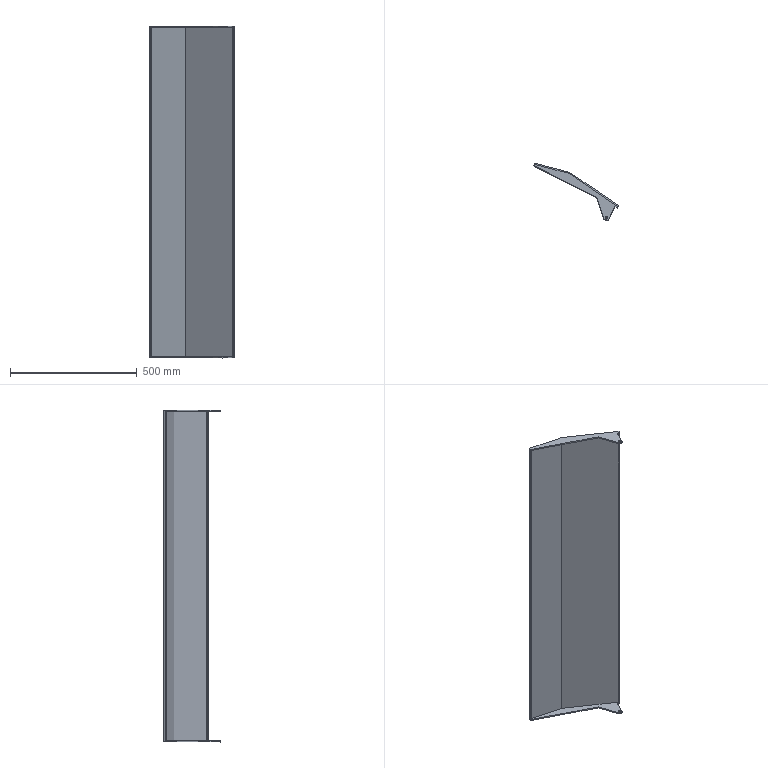Component | SolidWorks | SeedBoxTopCover-1 | 1 solid | 24 faces | box 334.55 x 225.9 x 1310 mm | volume 2630206 mm3 | plane 18 | cylinder 6 | commonest cylinder face diameters 10 x4 28.284 x2
build123d program:
from build123d import *

# Parameters (mm, degrees)
BOSS_EXTRUDE2_DEPTH = 1310
SHELL1_T            = -5
BOSS_EXTRUDE4_DEPTH = 5
SKETCH4_R           = 5
CUT_EXTRUDE1_DEPTH  = 1349.849


with BuildPart() as part:
    # Sketch1 → Boss-Extrude2 (new body)
    with BuildSketch(Plane.XY):
        Polygon((-54.92, 23.4), (-54.92, 33.4), (175.08, 63.4), (315.08, 33.4), (315.08, 23.4), (305.08, 23.4), (225.08, 23.4), align=None)
    extrude(amount=BOSS_EXTRUDE2_DEPTH)

    # Shell1
    shell1_openings = [part.faces().sort_by_distance(p)[0] for p in [
        (130.08, 23.4, 655),
    ]]
    offset(amount=SHELL1_T, openings=shell1_openings, kind=Kind.INTERSECTION)

    # Sketch3 → Boss-Extrude4 (add)
    with BuildSketch(Plane(origin=(0, 0, 0), x_dir=(-1, 0, 0), z_dir=(0, 0, -1))):
        with BuildLine():
            Line((-35.08, 23.4), (44.92, 23.4))
            Line((44.92, 23.4), (44.92, -36.6))
            ThreePointArc((44.92, -36.6), (34.92, -40.743), (24.92, -36.6))
            Line((24.92, -36.6), (-35.08, 23.4))
        make_face()
    boss_extrude4 = extrude(amount=-BOSS_EXTRUDE4_DEPTH)

    # Mirror2: Boss-Extrude4 across plane
    add(boss_extrude4.mirror(Plane.XY.offset(655)))

    # Sketch4 → Cut-Extrude1 (cut, through all)
    with BuildSketch(Plane(origin=(0, 0, 0), x_dir=(-1, 0, 0), z_dir=(0, 0, -1))):
        with Locations((34.92, -31.29)):
            Circle(SKETCH4_R)
    extrude(amount=-CUT_EXTRUDE1_DEPTH, mode=Mode.SUBTRACT)


solid = part.part

# Placed as in the assembly
solid = solid.moved(Location((466.915, -496.983, 2467.971), (-180, 0, -153.121)))
STEP:
#1=COLOUR_RGB('',0.7922,0.8196,0.9333);
#2=FILL_AREA_STYLE_COLOUR('',#1);
#3=FILL_AREA_STYLE('',(#2));
#4=SURFACE_STYLE_FILL_AREA(#3);
#5=SURFACE_SIDE_STYLE('',(#4));
#6=SURFACE_STYLE_USAGE(.BOTH.,#5);
#7=PRESENTATION_STYLE_ASSIGNMENT((#6));
#8=CARTESIAN_POINT('',(18.876,-21.198,45.589));
#9=VERTEX_POINT('',#8);
#10=CARTESIAN_POINT('',(19.227,-21.376,45.589));
#11=VERTEX_POINT('',#10);
#12=CARTESIAN_POINT('',(19.052,-21.287,45.589));
#13=DIRECTION('',(-0.,-0.,1.));
#14=DIRECTION('',(0.892,-0.4521,-0.));
#15=AXIS2_PLACEMENT_3D('',#12,#13,#14);
#16=CIRCLE('',#15,0.1969);
#17=EDGE_CURVE('',#9,#11,#16,.T.);
#18=ORIENTED_EDGE('',*,*,#17,.F.);
#19=CARTESIAN_POINT('',(18.876,-21.198,45.786));
#20=VERTEX_POINT('',#19);
#21=CARTESIAN_POINT('',(18.876,-21.198,45.589));
#22=DIRECTION('',(-0.,-0.,1.));
#23=VECTOR('',#22,39.37);
#24=LINE('',#21,#23);
#25=EDGE_CURVE('',#9,#20,#24,.T.);
#26=ORIENTED_EDGE('',*,*,#25,.T.);
#27=CARTESIAN_POINT('',(19.227,-21.376,45.786));
#28=VERTEX_POINT('',#27);
#29=CARTESIAN_POINT('',(19.052,-21.287,45.786));
#30=DIRECTION('',(-0.,-0.,1.));
#31=DIRECTION('',(0.892,-0.4521,-0.));
#32=AXIS2_PLACEMENT_3D('',#29,#30,#31);
#33=CIRCLE('',#32,0.1969);
#34=EDGE_CURVE('',#20,#28,#33,.T.);
#35=ORIENTED_EDGE('',*,*,#34,.T.);
#36=CARTESIAN_POINT('',(19.227,-21.376,45.589));
#37=DIRECTION('',(-0.,-0.,1.));
#38=VECTOR('',#37,39.37);
#39=LINE('',#36,#38);
#40=EDGE_CURVE('',#11,#28,#39,.T.);
#41=ORIENTED_EDGE('',*,*,#40,.F.);
#42=EDGE_LOOP('',(#18,#26,#35,#41));
#43=FACE_OUTER_BOUND('',#42,.T.);
#44=CARTESIAN_POINT('',(19.052,-21.287,45.589));
#45=DIRECTION('',(-0.,-0.,1.));
#46=DIRECTION('',(0.892,-0.4521,-0.));
#47=AXIS2_PLACEMENT_3D('',#44,#45,#46);
#48=CYLINDRICAL_SURFACE('',#47,0.1969);
#49=ADVANCED_FACE('',(#43),#48,.F.);
#50=CARTESIAN_POINT('',(18.876,-21.198,96.967));
#51=VERTEX_POINT('',#50);
#52=CARTESIAN_POINT('',(19.227,-21.376,96.967));
#53=VERTEX_POINT('',#52);
#54=CARTESIAN_POINT('',(19.052,-21.287,96.967));
#55=DIRECTION('',(-0.,-0.,1.));
#56=DIRECTION('',(0.892,-0.4521,-0.));
#57=AXIS2_PLACEMENT_3D('',#54,#55,#56);
#58=CIRCLE('',#57,0.1969);
#59=EDGE_CURVE('',#51,#53,#58,.T.);
#60=ORIENTED_EDGE('',*,*,#59,.F.);
#61=CARTESIAN_POINT('',(18.876,-21.198,97.164));
#62=VERTEX_POINT('',#61);
#63=CARTESIAN_POINT('',(18.876,-21.198,45.589));
#64=DIRECTION('',(-0.,-0.,1.));
#65=VECTOR('',#64,39.37);
#66=LINE('',#63,#65);
#67=EDGE_CURVE('',#51,#62,#66,.T.);
#68=ORIENTED_EDGE('',*,*,#67,.T.);
#69=CARTESIAN_POINT('',(19.227,-21.376,97.164));
#70=VERTEX_POINT('',#69);
#71=CARTESIAN_POINT('',(19.052,-21.287,97.164));
#72=DIRECTION('',(-0.,-0.,1.));
#73=DIRECTION('',(0.892,-0.4521,-0.));
#74=AXIS2_PLACEMENT_3D('',#71,#72,#73);
#75=CIRCLE('',#74,0.1969);
#76=EDGE_CURVE('',#62,#70,#75,.T.);
#77=ORIENTED_EDGE('',*,*,#76,.T.);
#78=CARTESIAN_POINT('',(19.227,-21.376,45.589));
#79=DIRECTION('',(-0.,-0.,1.));
#80=VECTOR('',#79,39.37);
#81=LINE('',#78,#80);
#82=EDGE_CURVE('',#53,#70,#81,.T.);
#83=ORIENTED_EDGE('',*,*,#82,.F.);
#84=EDGE_LOOP('',(#60,#68,#77,#83));
#85=FACE_OUTER_BOUND('',#84,.T.);
#86=CARTESIAN_POINT('',(19.052,-21.287,45.589));
#87=DIRECTION('',(-0.,-0.,1.));
#88=DIRECTION('',(0.892,-0.4521,-0.));
#89=AXIS2_PLACEMENT_3D('',#86,#87,#88);
#90=CYLINDRICAL_SURFACE('',#89,0.1969);
#91=ADVANCED_FACE('',(#85),#90,.F.);
#92=CARTESIAN_POINT('',(17.567,-18.12,45.786));
#93=VERTEX_POINT('',#92);
#94=CARTESIAN_POINT('',(17.567,-18.12,45.589));
#95=VERTEX_POINT('',#94);
#96=CARTESIAN_POINT('',(17.567,-18.12,45.786));
#97=DIRECTION('',(0.,0.,-1.));
#98=VECTOR('',#97,39.37);
#99=LINE('',#96,#98);
#100=EDGE_CURVE('',#93,#95,#99,.T.);
#101=ORIENTED_EDGE('',*,*,#100,.F.);
#102=CARTESIAN_POINT('',(7.91,-13.225,45.786));
#103=VERTEX_POINT('',#102);
#104=CARTESIAN_POINT('',(18.799,-18.745,45.786));
#105=DIRECTION('',(-0.892,0.4521,0.));
#106=VECTOR('',#105,39.37);
#107=LINE('',#104,#106);
#108=EDGE_CURVE('',#93,#103,#107,.T.);
#109=ORIENTED_EDGE('',*,*,#108,.T.);
#110=CARTESIAN_POINT('',(7.91,-13.225,96.967));
#111=VERTEX_POINT('',#110);
#112=CARTESIAN_POINT('',(7.91,-13.225,45.589));
#113=DIRECTION('',(-0.,-0.,1.));
#114=VECTOR('',#113,39.37);
#115=LINE('',#112,#114);
#116=EDGE_CURVE('',#103,#111,#115,.T.);
#117=ORIENTED_EDGE('',*,*,#116,.T.);
#118=CARTESIAN_POINT('',(17.567,-18.12,96.967));
#119=VERTEX_POINT('',#118);
#120=CARTESIAN_POINT('',(18.799,-18.745,96.967));
#121=DIRECTION('',(-0.892,0.4521,0.));
#122=VECTOR('',#121,39.37);
#123=LINE('',#120,#122);
#124=EDGE_CURVE('',#119,#111,#123,.T.);
#125=ORIENTED_EDGE('',*,*,#124,.F.);
#126=CARTESIAN_POINT('',(17.567,-18.12,97.164));
#127=VERTEX_POINT('',#126);
#128=CARTESIAN_POINT('',(17.567,-18.12,96.967));
#129=DIRECTION('',(-0.,-0.,1.));
#130=VECTOR('',#129,39.37);
#131=LINE('',#128,#130);
#132=EDGE_CURVE('',#119,#127,#131,.T.);
#133=ORIENTED_EDGE('',*,*,#132,.T.);
#134=CARTESIAN_POINT('',(7.734,-13.136,97.164));
#135=VERTEX_POINT('',#134);
#136=CARTESIAN_POINT('',(7.734,-13.136,97.164));
#137=DIRECTION('',(-0.892,0.4521,0.));
#138=VECTOR('',#137,39.37);
#139=LINE('',#136,#138);
#140=EDGE_CURVE('',#127,#135,#139,.T.);
#141=ORIENTED_EDGE('',*,*,#140,.T.);
#142=CARTESIAN_POINT('',(7.734,-13.136,45.589));
#143=VERTEX_POINT('',#142);
#144=CARTESIAN_POINT('',(7.734,-13.136,45.589));
#145=DIRECTION('',(-0.,-0.,1.));
#146=VECTOR('',#145,39.37);
#147=LINE('',#144,#146);
#148=EDGE_CURVE('',#143,#135,#147,.T.);
#149=ORIENTED_EDGE('',*,*,#148,.F.);
#150=CARTESIAN_POINT('',(20.728,-19.722,45.589));
#151=DIRECTION('',(-0.892,0.4521,0.));
#152=VECTOR('',#151,39.37);
#153=LINE('',#150,#152);
#154=EDGE_CURVE('',#95,#143,#153,.T.);
#155=ORIENTED_EDGE('',*,*,#154,.F.);
#156=EDGE_LOOP('',(#101,#109,#117,#125,#133,#141,#149,#155));
#157=FACE_OUTER_BOUND('',#156,.T.);
#158=CARTESIAN_POINT('',(7.734,-13.136,45.589));
#159=DIRECTION('',(0.4521,0.892,0.));
#160=DIRECTION('',(0.,0.,-1.));
#161=AXIS2_PLACEMENT_3D('',#158,#159,#160);
#162=PLANE('',#161);
#163=ADVANCED_FACE('',(#157),#162,.F.);
#164=CARTESIAN_POINT('',(20.376,-19.544,45.786));
#165=VERTEX_POINT('',#164);
#166=CARTESIAN_POINT('',(20.376,-19.544,45.589));
#167=VERTEX_POINT('',#166);
#168=CARTESIAN_POINT('',(20.376,-19.544,45.786));
#169=DIRECTION('',(0.,0.,-1.));
#170=VECTOR('',#169,39.37);
#171=LINE('',#168,#170);
#172=EDGE_CURVE('',#165,#167,#171,.T.);
#173=ORIENTED_EDGE('',*,*,#172,.T.);
#174=CARTESIAN_POINT('',(20.728,-19.722,45.589));
#175=VERTEX_POINT('',#174);
#176=CARTESIAN_POINT('',(20.728,-19.722,45.589));
#177=DIRECTION('',(-0.892,0.4521,0.));
#178=VECTOR('',#177,39.37);
#179=LINE('',#176,#178);
#180=EDGE_CURVE('',#175,#167,#179,.T.);
#181=ORIENTED_EDGE('',*,*,#180,.F.);
#182=CARTESIAN_POINT('',(20.728,-19.722,97.164));
#183=VERTEX_POINT('',#182);
#184=CARTESIAN_POINT('',(20.728,-19.722,45.589));
#185=DIRECTION('',(-0.,-0.,1.));
#186=VECTOR('',#185,39.37);
#187=LINE('',#184,#186);
#188=EDGE_CURVE('',#175,#183,#187,.T.);
#189=ORIENTED_EDGE('',*,*,#188,.T.);
#190=CARTESIAN_POINT('',(20.376,-19.544,97.164));
#191=VERTEX_POINT('',#190);
#192=CARTESIAN_POINT('',(7.734,-13.136,97.164));
#193=DIRECTION('',(-0.892,0.4521,0.));
#194=VECTOR('',#193,39.37);
#195=LINE('',#192,#194);
#196=EDGE_CURVE('',#183,#191,#195,.T.);
#197=ORIENTED_EDGE('',*,*,#196,.T.);
#198=CARTESIAN_POINT('',(20.376,-19.544,96.967));
#199=VERTEX_POINT('',#198);
#200=CARTESIAN_POINT('',(20.376,-19.544,96.967));
#201=DIRECTION('',(-0.,-0.,1.));
#202=VECTOR('',#201,39.37);
#203=LINE('',#200,#202);
#204=EDGE_CURVE('',#199,#191,#203,.T.);
#205=ORIENTED_EDGE('',*,*,#204,.F.);
#206=CARTESIAN_POINT('',(20.552,-19.633,96.967));
#207=VERTEX_POINT('',#206);
#208=CARTESIAN_POINT('',(18.799,-18.745,96.967));
#209=DIRECTION('',(-0.892,0.4521,0.));
#210=VECTOR('',#209,39.37);
#211=LINE('',#208,#210);
#212=EDGE_CURVE('',#207,#199,#211,.T.);
#213=ORIENTED_EDGE('',*,*,#212,.F.);
#214=CARTESIAN_POINT('',(20.552,-19.633,45.786));
#215=VERTEX_POINT('',#214);
#216=CARTESIAN_POINT('',(20.552,-19.633,45.589));
#217=DIRECTION('',(-0.,-0.,1.));
#218=VECTOR('',#217,39.37);
#219=LINE('',#216,#218);
#220=EDGE_CURVE('',#215,#207,#219,.T.);
#221=ORIENTED_EDGE('',*,*,#220,.F.);
#222=CARTESIAN_POINT('',(18.799,-18.745,45.786));
#223=DIRECTION('',(-0.892,0.4521,0.));
#224=VECTOR('',#223,39.37);
#225=LINE('',#222,#224);
#226=EDGE_CURVE('',#215,#165,#225,.T.);
#227=ORIENTED_EDGE('',*,*,#226,.T.);
#228=EDGE_LOOP('',(#173,#181,#189,#197,#205,#213,#221,#227));
#229=FACE_OUTER_BOUND('',#228,.T.);
#230=CARTESIAN_POINT('',(7.734,-13.136,45.589));
#231=DIRECTION('',(0.4521,0.892,0.));
#232=DIRECTION('',(0.,0.,-1.));
#233=AXIS2_PLACEMENT_3D('',#230,#231,#232);
#234=PLANE('',#233);
#235=ADVANCED_FACE('',(#229),#234,.F.);
#236=CARTESIAN_POINT('',(7.912,-12.785,97.164));
#237=VERTEX_POINT('',#236);
#238=CARTESIAN_POINT('',(7.912,-12.785,97.164));
#239=DIRECTION('',(0.4521,0.892,0.));
#240=VECTOR('',#239,39.37);
#241=LINE('',#238,#240);
#242=EDGE_CURVE('',#135,#237,#241,.T.);
#243=ORIENTED_EDGE('',*,*,#242,.T.);
#244=CARTESIAN_POINT('',(7.912,-12.785,45.589));
#245=VERTEX_POINT('',#244);
#246=CARTESIAN_POINT('',(7.912,-12.785,45.589));
#247=DIRECTION('',(-0.,-0.,1.));
#248=VECTOR('',#247,39.37);
#249=LINE('',#246,#248);
#250=EDGE_CURVE('',#245,#237,#249,.T.);
#251=ORIENTED_EDGE('',*,*,#250,.F.);
#252=CARTESIAN_POINT('',(7.912,-12.785,45.589));
#253=DIRECTION('',(0.4521,0.892,0.));
#254=VECTOR('',#253,39.37);
#255=LINE('',#252,#254);
#256=EDGE_CURVE('',#143,#245,#255,.T.);
#257=ORIENTED_EDGE('',*,*,#256,.F.);
#258=ORIENTED_EDGE('',*,*,#148,.T.);
#259=EDGE_LOOP('',(#243,#251,#257,#258));
#260=FACE_OUTER_BOUND('',#259,.T.);
#261=CARTESIAN_POINT('',(7.912,-12.785,45.589));
#262=DIRECTION('',(0.892,-0.4521,-0.));
#263=DIRECTION('',(0.,0.,-1.));
#264=AXIS2_PLACEMENT_3D('',#261,#262,#263);
#265=PLANE('',#264);
#266=ADVANCED_FACE('',(#260),#265,.F.);
#267=CARTESIAN_POINT('',(13.363,-14.224,97.164));
#268=VERTEX_POINT('',#267);
#269=CARTESIAN_POINT('',(13.363,-14.224,97.164));
#270=DIRECTION('',(0.9669,-0.2552,-0.));
#271=VECTOR('',#270,39.37);
#272=LINE('',#269,#271);
#273=EDGE_CURVE('',#237,#268,#272,.T.);
#274=ORIENTED_EDGE('',*,*,#273,.T.);
#275=CARTESIAN_POINT('',(13.363,-14.224,45.589));
#276=VERTEX_POINT('',#275);
#277=CARTESIAN_POINT('',(13.363,-14.224,45.589));
#278=DIRECTION('',(-0.,-0.,1.));
#279=VECTOR('',#278,39.37);
#280=LINE('',#277,#279);
#281=EDGE_CURVE('',#276,#268,#280,.T.);
#282=ORIENTED_EDGE('',*,*,#281,.F.);
#283=CARTESIAN_POINT('',(13.363,-14.224,45.589));
#284=DIRECTION('',(0.9669,-0.2552,-0.));
#285=VECTOR('',#284,39.37);
#286=LINE('',#283,#285);
#287=EDGE_CURVE('',#245,#276,#286,.T.);
#288=ORIENTED_EDGE('',*,*,#287,.F.);
#289=ORIENTED_EDGE('',*,*,#250,.T.);
#290=EDGE_LOOP('',(#274,#282,#288,#289));
#291=FACE_OUTER_BOUND('',#290,.T.);
#292=CARTESIAN_POINT('',(13.363,-14.224,45.589));
#293=DIRECTION('',(-0.2552,-0.9669,-0.));
#294=DIRECTION('',(-0.9669,0.2552,0.));
#295=AXIS2_PLACEMENT_3D('',#292,#293,#294);
#296=PLANE('',#295);
#297=ADVANCED_FACE('',(#291),#296,.F.);
#298=CARTESIAN_POINT('',(20.906,-19.371,97.164));
#299=VERTEX_POINT('',#298);
#300=CARTESIAN_POINT('',(13.363,-14.224,97.164));
#301=DIRECTION('',(0.826,-0.5637,-0.));
#302=VECTOR('',#301,39.37);
#303=LINE('',#300,#302);
#304=EDGE_CURVE('',#268,#299,#303,.T.);
#305=ORIENTED_EDGE('',*,*,#304,.T.);
#306=CARTESIAN_POINT('',(20.906,-19.371,45.589));
#307=VERTEX_POINT('',#306);
#308=CARTESIAN_POINT('',(20.906,-19.371,45.589));
#309=DIRECTION('',(-0.,-0.,1.));
#310=VECTOR('',#309,39.37);
#311=LINE('',#308,#310);
#312=EDGE_CURVE('',#307,#299,#311,.T.);
#313=ORIENTED_EDGE('',*,*,#312,.F.);
#314=CARTESIAN_POINT('',(13.363,-14.224,45.589));
#315=DIRECTION('',(0.826,-0.5637,-0.));
#316=VECTOR('',#315,39.37);
#317=LINE('',#314,#316);
#318=EDGE_CURVE('',#276,#307,#317,.T.);
#319=ORIENTED_EDGE('',*,*,#318,.F.);
#320=ORIENTED_EDGE('',*,*,#281,.T.);
#321=EDGE_LOOP('',(#305,#313,#319,#320));
#322=FACE_OUTER_BOUND('',#321,.T.);
#323=CARTESIAN_POINT('',(13.363,-14.224,45.589));
#324=DIRECTION('',(-0.5637,-0.826,-0.));
#325=DIRECTION('',(-0.826,0.5637,0.));
#326=AXIS2_PLACEMENT_3D('',#323,#324,#325);
#327=PLANE('',#326);
#328=ADVANCED_FACE('',(#322),#327,.F.);
#329=CARTESIAN_POINT('',(20.728,-19.722,97.164));
#330=DIRECTION('',(-0.4521,-0.892,-0.));
#331=VECTOR('',#330,39.37);
#332=LINE('',#329,#331);
#333=EDGE_CURVE('',#299,#183,#332,.T.);
#334=ORIENTED_EDGE('',*,*,#333,.T.);
#335=ORIENTED_EDGE('',*,*,#188,.F.);
#336=CARTESIAN_POINT('',(20.728,-19.722,45.589));
#337=DIRECTION('',(-0.4521,-0.892,-0.));
#338=VECTOR('',#337,39.37);
#339=LINE('',#336,#338);
#340=EDGE_CURVE('',#307,#175,#339,.T.);
#341=ORIENTED_EDGE('',*,*,#340,.F.);
#342=ORIENTED_EDGE('',*,*,#312,.T.);
#343=EDGE_LOOP('',(#334,#335,#341,#342));
#344=FACE_OUTER_BOUND('',#343,.T.);
#345=CARTESIAN_POINT('',(20.728,-19.722,45.589));
#346=DIRECTION('',(-0.892,0.4521,0.));
#347=DIRECTION('',(-0.,-0.,1.));
#348=AXIS2_PLACEMENT_3D('',#345,#346,#347);
#349=PLANE('',#348);
#350=ADVANCED_FACE('',(#344),#349,.F.);
#351=CARTESIAN_POINT('',(19.052,-21.287,45.589));
#352=DIRECTION('',(-0.,-0.,1.));
#353=DIRECTION('',(0.892,-0.4521,-0.));
#354=AXIS2_PLACEMENT_3D('',#351,#352,#353);
#355=CIRCLE('',#354,0.1969);
#356=EDGE_CURVE('',#11,#9,#355,.T.);
#357=ORIENTED_EDGE('',*,*,#356,.T.);
#358=ORIENTED_EDGE('',*,*,#17,.T.);
#359=EDGE_LOOP('',(#357,#358));
#360=FACE_BOUND('',#359,.T.);
#361=ORIENTED_EDGE('',*,*,#180,.T.);
#362=CARTESIAN_POINT('',(19.308,-21.651,45.589));
#363=VERTEX_POINT('',#362);
#364=CARTESIAN_POINT('',(20.376,-19.544,45.589));
#365=DIRECTION('',(0.4521,0.892,0.));
#366=VECTOR('',#365,39.37);
#367=LINE('',#364,#366);
#368=EDGE_CURVE('',#363,#167,#367,.T.);
#369=ORIENTED_EDGE('',*,*,#368,.F.);
#370=CARTESIAN_POINT('',(18.606,-21.295,45.589));
#371=VERTEX_POINT('',#370);
#372=CARTESIAN_POINT('',(19.135,-21.122,45.589));
#373=DIRECTION('',(-0.,-0.,1.));
#374=DIRECTION('',(0.892,-0.4521,-0.));
#375=AXIS2_PLACEMENT_3D('',#372,#373,#374);
#376=CIRCLE('',#375,0.5568);
#377=EDGE_CURVE('',#371,#363,#376,.T.);
#378=ORIENTED_EDGE('',*,*,#377,.F.);
#379=CARTESIAN_POINT('',(18.606,-21.295,45.589));
#380=DIRECTION('',(0.311,-0.9504,-0.));
#381=VECTOR('',#380,39.37);
#382=LINE('',#379,#381);
#383=EDGE_CURVE('',#95,#371,#382,.T.);
#384=ORIENTED_EDGE('',*,*,#383,.F.);
#385=ORIENTED_EDGE('',*,*,#154,.T.);
#386=ORIENTED_EDGE('',*,*,#256,.T.);
#387=ORIENTED_EDGE('',*,*,#287,.T.);
#388=ORIENTED_EDGE('',*,*,#318,.T.);
#389=ORIENTED_EDGE('',*,*,#340,.T.);
#390=EDGE_LOOP('',(#361,#369,#378,#384,#385,#386,#387,#388,#389));
#391=FACE_OUTER_BOUND('',#390,.T.);
#392=CARTESIAN_POINT('',(18.382,-19.566,45.589));
#393=DIRECTION('',(-0.,-0.,1.));
#394=DIRECTION('',(0.892,-0.4521,-0.));
#395=AXIS2_PLACEMENT_3D('',#392,#393,#394);
#396=PLANE('',#395);
#397=ADVANCED_FACE('',(#360,#391),#396,.F.);
#398=CARTESIAN_POINT('',(19.052,-21.287,97.164));
#399=DIRECTION('',(-0.,-0.,1.));
#400=DIRECTION('',(0.892,-0.4521,-0.));
#401=AXIS2_PLACEMENT_3D('',#398,#399,#400);
#402=CIRCLE('',#401,0.1969);
#403=EDGE_CURVE('',#70,#62,#402,.T.);
#404=ORIENTED_EDGE('',*,*,#403,.F.);
#405=ORIENTED_EDGE('',*,*,#76,.F.);
#406=EDGE_LOOP('',(#404,#405));
#407=FACE_BOUND('',#406,.T.);
#408=ORIENTED_EDGE('',*,*,#196,.F.);
#409=ORIENTED_EDGE('',*,*,#333,.F.);
#410=ORIENTED_EDGE('',*,*,#304,.F.);
#411=ORIENTED_EDGE('',*,*,#273,.F.);
#412=ORIENTED_EDGE('',*,*,#242,.F.);
#413=ORIENTED_EDGE('',*,*,#140,.F.);
#414=CARTESIAN_POINT('',(18.606,-21.295,97.164));
#415=VERTEX_POINT('',#414);
#416=CARTESIAN_POINT('',(18.606,-21.295,97.164));
#417=DIRECTION('',(0.311,-0.9504,-0.));
#418=VECTOR('',#417,39.37);
#419=LINE('',#416,#418);
#420=EDGE_CURVE('',#127,#415,#419,.T.);
#421=ORIENTED_EDGE('',*,*,#420,.T.);
#422=CARTESIAN_POINT('',(19.308,-21.651,97.164));
#423=VERTEX_POINT('',#422);
#424=CARTESIAN_POINT('',(19.135,-21.122,97.164));
#425=DIRECTION('',(-0.,-0.,1.));
#426=DIRECTION('',(0.892,-0.4521,-0.));
#427=AXIS2_PLACEMENT_3D('',#424,#425,#426);
#428=CIRCLE('',#427,0.5568);
#429=EDGE_CURVE('',#415,#423,#428,.T.);
#430=ORIENTED_EDGE('',*,*,#429,.T.);
#431=CARTESIAN_POINT('',(20.376,-19.544,97.164));
#432=DIRECTION('',(0.4521,0.892,0.));
#433=VECTOR('',#432,39.37);
#434=LINE('',#431,#433);
#435=EDGE_CURVE('',#423,#191,#434,.T.);
#436=ORIENTED_EDGE('',*,*,#435,.T.);
#437=EDGE_LOOP('',(#408,#409,#410,#411,#412,#413,#421,#430,#436));
#438=FACE_OUTER_BOUND('',#437,.T.);
#439=CARTESIAN_POINT('',(18.382,-19.566,97.164));
#440=DIRECTION('',(-0.,-0.,1.));
#441=DIRECTION('',(0.892,-0.4521,-0.));
#442=AXIS2_PLACEMENT_3D('',#439,#440,#441);
#443=PLANE('',#442);
#444=ADVANCED_FACE('',(#407,#438),#443,.T.);
#445=CARTESIAN_POINT('',(8.016,-13.016,96.967));
#446=VERTEX_POINT('',#445);
#447=CARTESIAN_POINT('',(7.493,-14.047,96.967));
#448=DIRECTION('',(0.4521,0.892,0.));
#449=VECTOR('',#448,39.37);
#450=LINE('',#447,#449);
#451=EDGE_CURVE('',#111,#446,#450,.T.);
#452=ORIENTED_EDGE('',*,*,#451,.F.);
#453=ORIENTED_EDGE('',*,*,#116,.F.);
#454=CARTESIAN_POINT('',(8.016,-13.016,45.786));
#455=VERTEX_POINT('',#454);
#456=CARTESIAN_POINT('',(7.493,-14.047,45.786));
#457=DIRECTION('',(0.4521,0.892,0.));
#458=VECTOR('',#457,39.37);
#459=LINE('',#456,#458);
#460=EDGE_CURVE('',#103,#455,#459,.T.);
#461=ORIENTED_EDGE('',*,*,#460,.T.);
#462=CARTESIAN_POINT('',(8.016,-13.016,45.589));
#463=DIRECTION('',(-0.,-0.,1.));
#464=VECTOR('',#463,39.37);
#465=LINE('',#462,#464);
#466=EDGE_CURVE('',#455,#446,#465,.T.);
#467=ORIENTED_EDGE('',*,*,#466,.T.);
#468=EDGE_LOOP('',(#452,#453,#461,#467));
#469=FACE_OUTER_BOUND('',#468,.T.);
#470=CARTESIAN_POINT('',(8.088,-12.874,45.589));
#471=DIRECTION('',(0.892,-0.4521,-0.));
#472=DIRECTION('',(0.,0.,-1.));
#473=AXIS2_PLACEMENT_3D('',#470,#471,#472);
#474=PLANE('',#473);
#475=ADVANCED_FACE('',(#469),#474,.T.);
#476=CARTESIAN_POINT('',(13.28,-14.405,96.967));
#477=VERTEX_POINT('',#476);
#478=CARTESIAN_POINT('',(19.324,-16.,96.967));
#479=DIRECTION('',(0.9669,-0.2552,-0.));
#480=VECTOR('',#479,39.37);
#481=LINE('',#478,#480);
#482=EDGE_CURVE('',#446,#477,#481,.T.);
#483=ORIENTED_EDGE('',*,*,#482,.F.);
#484=ORIENTED_EDGE('',*,*,#466,.F.);
#485=CARTESIAN_POINT('',(13.28,-14.405,45.786));
#486=VERTEX_POINT('',#485);
#487=CARTESIAN_POINT('',(19.324,-16.,45.786));
#488=DIRECTION('',(0.9669,-0.2552,-0.));
#489=VECTOR('',#488,39.37);
#490=LINE('',#487,#489);
#491=EDGE_CURVE('',#455,#486,#490,.T.);
#492=ORIENTED_EDGE('',*,*,#491,.T.);
#493=CARTESIAN_POINT('',(13.28,-14.405,45.589));
#494=DIRECTION('',(-0.,-0.,1.));
#495=VECTOR('',#494,39.37);
#496=LINE('',#493,#495);
#497=EDGE_CURVE('',#486,#477,#496,.T.);
#498=ORIENTED_EDGE('',*,*,#497,.T.);
#499=EDGE_LOOP('',(#483,#484,#492,#498));
#500=FACE_OUTER_BOUND('',#499,.T.);
#501=CARTESIAN_POINT('',(13.312,-14.414,45.589));
#502=DIRECTION('',(-0.2552,-0.9669,-0.));
#503=DIRECTION('',(-0.9669,0.2552,0.));
#504=AXIS2_PLACEMENT_3D('',#501,#502,#503);
#505=PLANE('',#504);
#506=ADVANCED_FACE('',(#500),#505,.T.);
#507=CARTESIAN_POINT('',(20.652,-19.436,96.967));
#508=VERTEX_POINT('',#507);
#509=CARTESIAN_POINT('',(19.164,-18.421,96.967));
#510=DIRECTION('',(0.826,-0.5637,-0.));
#511=VECTOR('',#510,39.37);
#512=LINE('',#509,#511);
#513=EDGE_CURVE('',#477,#508,#512,.T.);
#514=ORIENTED_EDGE('',*,*,#513,.F.);
#515=ORIENTED_EDGE('',*,*,#497,.F.);
#516=CARTESIAN_POINT('',(20.652,-19.436,45.786));
#517=VERTEX_POINT('',#516);
#518=CARTESIAN_POINT('',(19.164,-18.421,45.786));
#519=DIRECTION('',(0.826,-0.5637,-0.));
#520=VECTOR('',#519,39.37);
#521=LINE('',#518,#520);
#522=EDGE_CURVE('',#486,#517,#521,.T.);
#523=ORIENTED_EDGE('',*,*,#522,.T.);
#524=CARTESIAN_POINT('',(20.652,-19.436,45.589));
#525=DIRECTION('',(-0.,-0.,1.));
#526=VECTOR('',#525,39.37);
#527=LINE('',#524,#526);
#528=EDGE_CURVE('',#517,#508,#527,.T.);
#529=ORIENTED_EDGE('',*,*,#528,.T.);
#530=EDGE_LOOP('',(#514,#515,#523,#529));
#531=FACE_OUTER_BOUND('',#530,.T.);
#532=CARTESIAN_POINT('',(13.252,-14.386,45.589));
#533=DIRECTION('',(-0.5637,-0.826,-0.));
#534=DIRECTION('',(-0.826,0.5637,0.));
#535=AXIS2_PLACEMENT_3D('',#532,#533,#534);
#536=PLANE('',#535);
#537=ADVANCED_FACE('',(#531),#536,.T.);
#538=CARTESIAN_POINT('',(20.136,-20.455,96.967));
#539=DIRECTION('',(-0.4521,-0.892,-0.));
#540=VECTOR('',#539,39.37);
#541=LINE('',#538,#540);
#542=EDGE_CURVE('',#508,#207,#541,.T.);
#543=ORIENTED_EDGE('',*,*,#542,.F.);
#544=ORIENTED_EDGE('',*,*,#528,.F.);
#545=CARTESIAN_POINT('',(20.136,-20.455,45.786));
#546=DIRECTION('',(-0.4521,-0.892,-0.));
#547=VECTOR('',#546,39.37);
#548=LINE('',#545,#547);
#549=EDGE_CURVE('',#517,#215,#548,.T.);
#550=ORIENTED_EDGE('',*,*,#549,.T.);
#551=ORIENTED_EDGE('',*,*,#220,.T.);
#552=EDGE_LOOP('',(#543,#544,#550,#551));
#553=FACE_OUTER_BOUND('',#552,.T.);
#554=CARTESIAN_POINT('',(20.552,-19.633,45.589));
#555=DIRECTION('',(-0.892,0.4521,0.));
#556=DIRECTION('',(-0.,-0.,1.));
#557=AXIS2_PLACEMENT_3D('',#554,#555,#556);
#558=PLANE('',#557);
#559=ADVANCED_FACE('',(#553),#558,.T.);
#560=CARTESIAN_POINT('',(19.052,-21.287,45.786));
#561=DIRECTION('',(-0.,-0.,1.));
#562=DIRECTION('',(0.892,-0.4521,-0.));
#563=AXIS2_PLACEMENT_3D('',#560,#561,#562);
#564=CIRCLE('',#563,0.1969);
#565=EDGE_CURVE('',#28,#20,#564,.T.);
#566=ORIENTED_EDGE('',*,*,#565,.F.);
#567=ORIENTED_EDGE('',*,*,#34,.F.);
#568=EDGE_LOOP('',(#566,#567));
#569=FACE_BOUND('',#568,.T.);
#570=ORIENTED_EDGE('',*,*,#226,.F.);
#571=ORIENTED_EDGE('',*,*,#549,.F.);
#572=ORIENTED_EDGE('',*,*,#522,.F.);
#573=ORIENTED_EDGE('',*,*,#491,.F.);
#574=ORIENTED_EDGE('',*,*,#460,.F.);
#575=ORIENTED_EDGE('',*,*,#108,.F.);
#576=CARTESIAN_POINT('',(18.606,-21.295,45.786));
#577=VERTEX_POINT('',#576);
#578=CARTESIAN_POINT('',(18.606,-21.295,45.786));
#579=DIRECTION('',(0.311,-0.9504,-0.));
#580=VECTOR('',#579,39.37);
#581=LINE('',#578,#580);
#582=EDGE_CURVE('',#93,#577,#581,.T.);
#583=ORIENTED_EDGE('',*,*,#582,.T.);
#584=CARTESIAN_POINT('',(19.308,-21.651,45.786));
#585=VERTEX_POINT('',#584);
#586=CARTESIAN_POINT('',(19.135,-21.122,45.786));
#587=DIRECTION('',(-0.,-0.,1.));
#588=DIRECTION('',(0.892,-0.4521,-0.));
#589=AXIS2_PLACEMENT_3D('',#586,#587,#588);
#590=CIRCLE('',#589,0.5568);
#591=EDGE_CURVE('',#577,#585,#590,.T.);
#592=ORIENTED_EDGE('',*,*,#591,.T.);
#593=CARTESIAN_POINT('',(20.376,-19.544,45.786));
#594=DIRECTION('',(0.4521,0.892,0.));
#595=VECTOR('',#594,39.37);
#596=LINE('',#593,#595);
#597=EDGE_CURVE('',#585,#165,#596,.T.);
#598=ORIENTED_EDGE('',*,*,#597,.T.);
#599=EDGE_LOOP('',(#570,#571,#572,#573,#574,#575,#583,#592,#598));
#600=FACE_OUTER_BOUND('',#599,.T.);
#601=CARTESIAN_POINT('',(18.382,-19.566,45.786));
#602=DIRECTION('',(-0.,-0.,1.));
#603=DIRECTION('',(0.892,-0.4521,-0.));
#604=AXIS2_PLACEMENT_3D('',#601,#602,#603);
#605=PLANE('',#604);
#606=ADVANCED_FACE('',(#569,#600),#605,.T.);
#607=CARTESIAN_POINT('',(19.052,-21.287,96.967));
#608=DIRECTION('',(-0.,-0.,1.));
#609=DIRECTION('',(0.892,-0.4521,-0.));
#610=AXIS2_PLACEMENT_3D('',#607,#608,#609);
#611=CIRCLE('',#610,0.1969);
#612=EDGE_CURVE('',#53,#51,#611,.T.);
#613=ORIENTED_EDGE('',*,*,#612,.T.);
#614=ORIENTED_EDGE('',*,*,#59,.T.);
#615=EDGE_LOOP('',(#613,#614));
#616=FACE_BOUND('',#615,.T.);
#617=ORIENTED_EDGE('',*,*,#212,.T.);
#618=CARTESIAN_POINT('',(19.308,-21.651,96.967));
#619=VERTEX_POINT('',#618);
#620=CARTESIAN_POINT('',(20.376,-19.544,96.967));
#621=DIRECTION('',(0.4521,0.892,0.));
#622=VECTOR('',#621,39.37);
#623=LINE('',#620,#622);
#624=EDGE_CURVE('',#619,#199,#623,.T.);
#625=ORIENTED_EDGE('',*,*,#624,.F.);
#626=CARTESIAN_POINT('',(18.606,-21.295,96.967));
#627=VERTEX_POINT('',#626);
#628=CARTESIAN_POINT('',(19.135,-21.122,96.967));
#629=DIRECTION('',(-0.,-0.,1.));
#630=DIRECTION('',(0.892,-0.4521,-0.));
#631=AXIS2_PLACEMENT_3D('',#628,#629,#630);
#632=CIRCLE('',#631,0.5568);
#633=EDGE_CURVE('',#627,#619,#632,.T.);
#634=ORIENTED_EDGE('',*,*,#633,.F.);
#635=CARTESIAN_POINT('',(18.606,-21.295,96.967));
#636=DIRECTION('',(0.311,-0.9504,-0.));
#637=VECTOR('',#636,39.37);
#638=LINE('',#635,#637);
#639=EDGE_CURVE('',#119,#627,#638,.T.);
#640=ORIENTED_EDGE('',*,*,#639,.F.);
#641=ORIENTED_EDGE('',*,*,#124,.T.);
#642=ORIENTED_EDGE('',*,*,#451,.T.);
#643=ORIENTED_EDGE('',*,*,#482,.T.);
#644=ORIENTED_EDGE('',*,*,#513,.T.);
#645=ORIENTED_EDGE('',*,*,#542,.T.);
#646=EDGE_LOOP('',(#617,#625,#634,#640,#641,#642,#643,#644,#645));
#647=FACE_OUTER_BOUND('',#646,.T.);
#648=CARTESIAN_POINT('',(18.382,-19.566,96.967));
#649=DIRECTION('',(-0.,-0.,1.));
#650=DIRECTION('',(0.892,-0.4521,-0.));
#651=AXIS2_PLACEMENT_3D('',#648,#649,#650);
#652=PLANE('',#651);
#653=ADVANCED_FACE('',(#616,#647),#652,.F.);
#654=ORIENTED_EDGE('',*,*,#420,.F.);
#655=ORIENTED_EDGE('',*,*,#132,.F.);
#656=ORIENTED_EDGE('',*,*,#639,.T.);
#657=CARTESIAN_POINT('',(18.606,-21.295,96.967));
#658=DIRECTION('',(-0.,-0.,1.));
#659=VECTOR('',#658,39.37);
#660=LINE('',#657,#659);
#661=EDGE_CURVE('',#627,#415,#660,.T.);
#662=ORIENTED_EDGE('',*,*,#661,.T.);
#663=EDGE_LOOP('',(#654,#655,#656,#662));
#664=FACE_OUTER_BOUND('',#663,.T.);
#665=CARTESIAN_POINT('',(18.606,-21.295,96.967));
#666=DIRECTION('',(-0.9504,-0.311,-0.));
#667=DIRECTION('',(-0.311,0.9504,0.));
#668=AXIS2_PLACEMENT_3D('',#665,#666,#667);
#669=PLANE('',#668);
#670=ADVANCED_FACE('',(#664),#669,.T.);
#671=ORIENTED_EDGE('',*,*,#435,.F.);
#672=CARTESIAN_POINT('',(19.308,-21.651,96.967));
#673=DIRECTION('',(-0.,-0.,1.));
#674=VECTOR('',#673,39.37);
#675=LINE('',#672,#674);
#676=EDGE_CURVE('',#619,#423,#675,.T.);
#677=ORIENTED_EDGE('',*,*,#676,.F.);
#678=ORIENTED_EDGE('',*,*,#624,.T.);
#679=ORIENTED_EDGE('',*,*,#204,.T.);
#680=EDGE_LOOP('',(#671,#677,#678,#679));
#681=FACE_OUTER_BOUND('',#680,.T.);
#682=CARTESIAN_POINT('',(20.376,-19.544,96.967));
#683=DIRECTION('',(0.892,-0.4521,-0.));
#684=DIRECTION('',(-0.4521,-0.892,-0.));
#685=AXIS2_PLACEMENT_3D('',#682,#683,#684);
#686=PLANE('',#685);
#687=ADVANCED_FACE('',(#681),#686,.T.);
#688=ORIENTED_EDGE('',*,*,#429,.F.);
#689=ORIENTED_EDGE('',*,*,#661,.F.);
#690=ORIENTED_EDGE('',*,*,#633,.T.);
#691=ORIENTED_EDGE('',*,*,#676,.T.);
#692=EDGE_LOOP('',(#688,#689,#690,#691));
#693=FACE_OUTER_BOUND('',#692,.T.);
#694=CARTESIAN_POINT('',(19.135,-21.122,96.967));
#695=DIRECTION('',(-0.,-0.,1.));
#696=DIRECTION('',(0.892,-0.4521,-0.));
#697=AXIS2_PLACEMENT_3D('',#694,#695,#696);
#698=CYLINDRICAL_SURFACE('',#697,0.5568);
#699=ADVANCED_FACE('',(#693),#698,.T.);
#700=ORIENTED_EDGE('',*,*,#383,.T.);
#701=CARTESIAN_POINT('',(18.606,-21.295,45.786));
#702=DIRECTION('',(0.,0.,-1.));
#703=VECTOR('',#702,39.37);
#704=LINE('',#701,#703);
#705=EDGE_CURVE('',#577,#371,#704,.T.);
#706=ORIENTED_EDGE('',*,*,#705,.F.);
#707=ORIENTED_EDGE('',*,*,#582,.F.);
#708=ORIENTED_EDGE('',*,*,#100,.T.);
#709=EDGE_LOOP('',(#700,#706,#707,#708));
#710=FACE_OUTER_BOUND('',#709,.T.);
#711=CARTESIAN_POINT('',(18.606,-21.295,45.786));
#712=DIRECTION('',(0.9504,0.311,0.));
#713=DIRECTION('',(0.311,-0.9504,-0.));
#714=AXIS2_PLACEMENT_3D('',#711,#712,#713);
#715=PLANE('',#714);
#716=ADVANCED_FACE('',(#710),#715,.F.);
#717=ORIENTED_EDGE('',*,*,#377,.T.);
#718=CARTESIAN_POINT('',(19.308,-21.651,45.786));
#719=DIRECTION('',(0.,0.,-1.));
#720=VECTOR('',#719,39.37);
#721=LINE('',#718,#720);
#722=EDGE_CURVE('',#585,#363,#721,.T.);
#723=ORIENTED_EDGE('',*,*,#722,.F.);
#724=ORIENTED_EDGE('',*,*,#591,.F.);
#725=ORIENTED_EDGE('',*,*,#705,.T.);
#726=EDGE_LOOP('',(#717,#723,#724,#725));
#727=FACE_OUTER_BOUND('',#726,.T.);
#728=CARTESIAN_POINT('',(19.135,-21.122,45.786));
#729=DIRECTION('',(0.,0.,-1.));
#730=DIRECTION('',(-0.892,0.4521,0.));
#731=AXIS2_PLACEMENT_3D('',#728,#729,#730);
#732=CYLINDRICAL_SURFACE('',#731,0.5568);
#733=ADVANCED_FACE('',(#727),#732,.T.);
#734=ORIENTED_EDGE('',*,*,#368,.T.);
#735=ORIENTED_EDGE('',*,*,#172,.F.);
#736=ORIENTED_EDGE('',*,*,#597,.F.);
#737=ORIENTED_EDGE('',*,*,#722,.T.);
#738=EDGE_LOOP('',(#734,#735,#736,#737));
#739=FACE_OUTER_BOUND('',#738,.T.);
#740=CARTESIAN_POINT('',(20.376,-19.544,45.786));
#741=DIRECTION('',(-0.892,0.4521,0.));
#742=DIRECTION('',(0.4521,0.892,0.));
#743=AXIS2_PLACEMENT_3D('',#740,#741,#742);
#744=PLANE('',#743);
#745=ADVANCED_FACE('',(#739),#744,.F.);
#746=ORIENTED_EDGE('',*,*,#67,.F.);
#747=ORIENTED_EDGE('',*,*,#612,.F.);
#748=ORIENTED_EDGE('',*,*,#82,.T.);
#749=ORIENTED_EDGE('',*,*,#403,.T.);
#750=EDGE_LOOP('',(#746,#747,#748,#749));
#751=FACE_OUTER_BOUND('',#750,.T.);
#752=CARTESIAN_POINT('',(19.052,-21.287,45.589));
#753=DIRECTION('',(-0.,-0.,1.));
#754=DIRECTION('',(0.892,-0.4521,-0.));
#755=AXIS2_PLACEMENT_3D('',#752,#753,#754);
#756=CYLINDRICAL_SURFACE('',#755,0.1969);
#757=ADVANCED_FACE('',(#751),#756,.F.);
#758=ORIENTED_EDGE('',*,*,#25,.F.);
#759=ORIENTED_EDGE('',*,*,#356,.F.);
#760=ORIENTED_EDGE('',*,*,#40,.T.);
#761=ORIENTED_EDGE('',*,*,#565,.T.);
#762=EDGE_LOOP('',(#758,#759,#760,#761));
#763=FACE_OUTER_BOUND('',#762,.T.);
#764=CARTESIAN_POINT('',(19.052,-21.287,45.589));
#765=DIRECTION('',(-0.,-0.,1.));
#766=DIRECTION('',(0.892,-0.4521,-0.));
#767=AXIS2_PLACEMENT_3D('',#764,#765,#766);
#768=CYLINDRICAL_SURFACE('',#767,0.1969);
#769=ADVANCED_FACE('',(#763),#768,.F.);
#770=CLOSED_SHELL('',(#49,#91,#163,#235,#266,#297,#328,#350,#397,#444,#475,#506,#537,#559,#606,#653,#670,#687,#699,#716,#733,#745,#757,#769));
#771=MANIFOLD_SOLID_BREP('',#770);
#772=STYLED_ITEM('',(#7),#771);
#773=(LENGTH_UNIT()NAMED_UNIT(*)SI_UNIT($,.METRE.));
#774=LENGTH_MEASURE_WITH_UNIT(LENGTH_MEASURE(0.0254),#773);
#775=DIMENSIONAL_EXPONENTS(1.,0.,0.,0.,0.,0.,0.);
#776=(CONVERSION_BASED_UNIT('',#774)LENGTH_UNIT()NAMED_UNIT(#775));
#777=UNCERTAINTY_MEASURE_WITH_UNIT(LENGTH_MEASURE(0.00001),#776,'','');
#778=(NAMED_UNIT(*)PLANE_ANGLE_UNIT()SI_UNIT($,.RADIAN.));
#779=(NAMED_UNIT(*)SI_UNIT($,.STERADIAN.)SOLID_ANGLE_UNIT());
#780=(GEOMETRIC_REPRESENTATION_CONTEXT(3)GLOBAL_UNCERTAINTY_ASSIGNED_CONTEXT((#777))GLOBAL_UNIT_ASSIGNED_CONTEXT((#776,#778,#779))REPRESENTATION_CONTEXT('',''));
#781=MECHANICAL_DESIGN_GEOMETRIC_PRESENTATION_REPRESENTATION('',(#772),#780);
#782=PRESENTATION_LAYER_ASSIGNMENT('','',(#772));
#783=CARTESIAN_POINT('',(0.,0.,0.));
#784=DIRECTION('',(0.,0.,1.));
#785=DIRECTION('',(1.,0.,0.));
#786=AXIS2_PLACEMENT_3D('',#783,#784,#785);
#787=(LENGTH_UNIT()NAMED_UNIT(*)SI_UNIT($,.METRE.));
#788=LENGTH_MEASURE_WITH_UNIT(LENGTH_MEASURE(0.0254),#787);
#789=DIMENSIONAL_EXPONENTS(1.,0.,0.,0.,0.,0.,0.);
#790=(CONVERSION_BASED_UNIT('',#788)LENGTH_UNIT()NAMED_UNIT(#789));
#791=UNCERTAINTY_MEASURE_WITH_UNIT(LENGTH_MEASURE(0.00001),#790,'','');
#792=(NAMED_UNIT(*)PLANE_ANGLE_UNIT()SI_UNIT($,.RADIAN.));
#793=(NAMED_UNIT(*)SI_UNIT($,.STERADIAN.)SOLID_ANGLE_UNIT());
#794=(GEOMETRIC_REPRESENTATION_CONTEXT(3)GLOBAL_UNCERTAINTY_ASSIGNED_CONTEXT((#791))GLOBAL_UNIT_ASSIGNED_CONTEXT((#790,#792,#793))REPRESENTATION_CONTEXT('',''));
#795=ADVANCED_BREP_SHAPE_REPRESENTATION('',(#771,#786),#794);